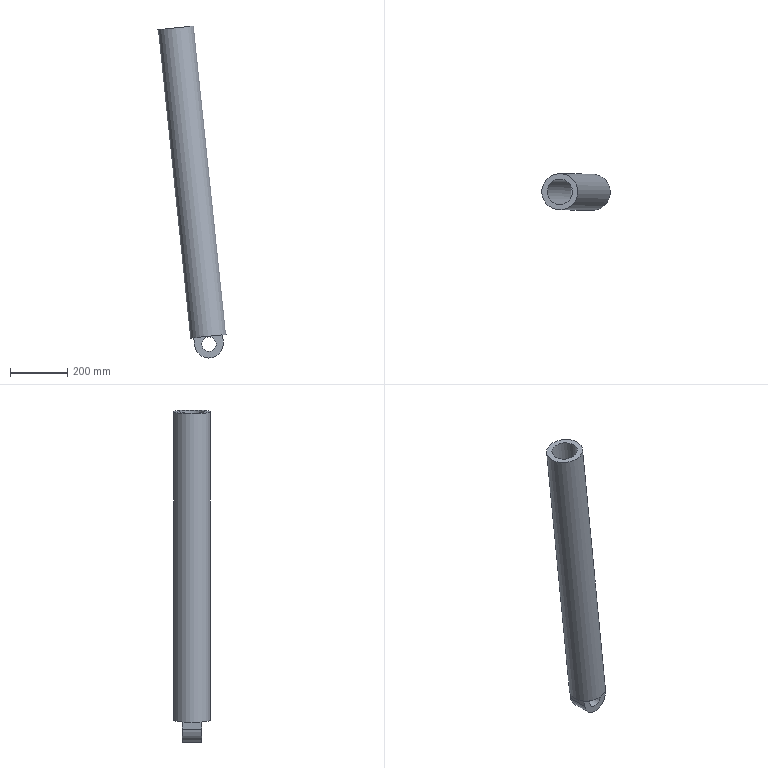Component | NX | LARGE_ARM_CYL_BODY_2 | 1 solid | 11 faces | volume 9202709 mm3 | plane 7 | cylinder 4 | commonest cylinder face diameters 127 x1 89 x1 101.6 x1 50.8 x1